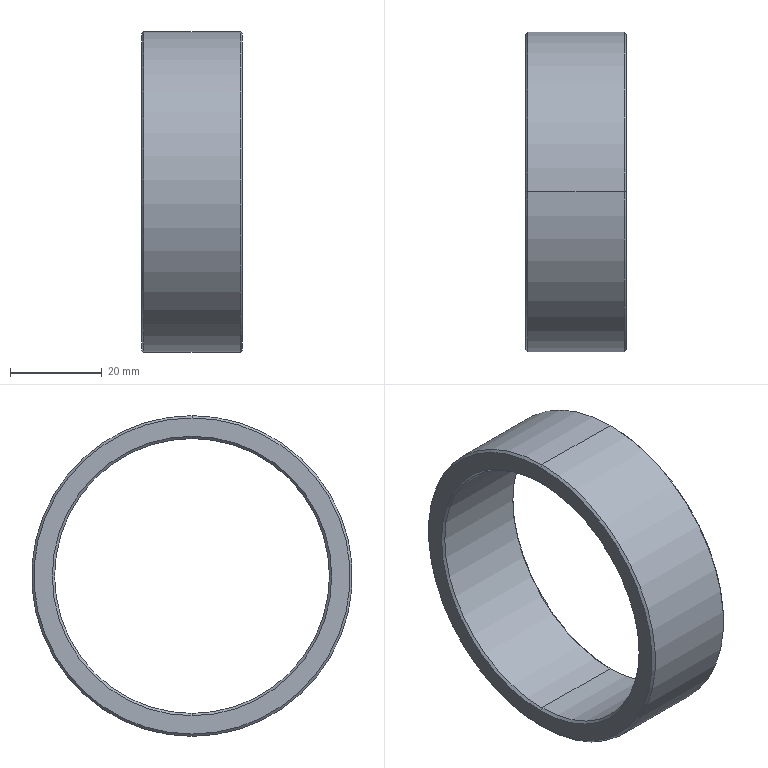Component | SolidWorks | Oil-impregnatedBushing-1 | 1 solid | 14 faces | box 22 x 70 x 70 mm | volume 22360 mm3 | cone 8 | cylinder 4 | plane 2 | commonest cylinder face diameters 60 x2 70 x2
build123d program:
from build123d import *

# Parameters (mm, degrees)
SKETCH1_R           = 35
SKETCH1_R_2         = 30
BOSS_EXTRUDE1_DEPTH = 22
CHAMFER1_SIZE       = 0.5


with BuildPart() as part:
    # Sketch1 → Boss-Extrude1 (new body)
    with BuildSketch(Plane.XY):
        Circle(SKETCH1_R)
        Circle(SKETCH1_R_2, mode=Mode.SUBTRACT)
    extrude(amount=BOSS_EXTRUDE1_DEPTH)

    # Chamfer1
    chamfer1_edges = [part.edges().sort_by_distance(p)[0] for p in [
        (-35, 0, 0),
        (-35, 0, 22),
        (-30, 0, 0),
        (-30, 0, 22),
    ]]
    chamfer(chamfer1_edges, length=CHAMFER1_SIZE)


solid = part.part

# Placed as in the assembly
solid = solid.moved(Location((-477.809, 275.819, 0), (0, 90, 0)))
STEP:
#1=COLOUR_RGB('',0.7922,0.8196,0.9333);
#2=FILL_AREA_STYLE_COLOUR('',#1);
#3=FILL_AREA_STYLE('',(#2));
#4=SURFACE_STYLE_FILL_AREA(#3);
#5=SURFACE_SIDE_STYLE('',(#4));
#6=SURFACE_STYLE_USAGE(.BOTH.,#5);
#7=PRESENTATION_STYLE_ASSIGNMENT((#6));
#8=CARTESIAN_POINT('',(-17.965,10.859,1.181));
#9=VERTEX_POINT('',#8);
#10=CARTESIAN_POINT('',(-17.965,10.859,-1.181));
#11=VERTEX_POINT('',#10);
#12=CARTESIAN_POINT('',(-17.965,10.859,0.));
#13=DIRECTION('',(1.,0.,0.));
#14=DIRECTION('',(0.,0.,-1.));
#15=AXIS2_PLACEMENT_3D('',#12,#13,#14);
#16=CIRCLE('',#15,1.181);
#17=EDGE_CURVE('',#9,#11,#16,.T.);
#18=ORIENTED_EDGE('',*,*,#17,.F.);
#19=CARTESIAN_POINT('',(-17.945,10.859,1.201));
#20=VERTEX_POINT('',#19);
#21=CARTESIAN_POINT('',(-17.965,10.859,1.181));
#22=DIRECTION('',(0.7071,0.,0.7071));
#23=VECTOR('',#22,39.37);
#24=LINE('',#21,#23);
#25=EDGE_CURVE('',#9,#20,#24,.T.);
#26=ORIENTED_EDGE('',*,*,#25,.T.);
#27=CARTESIAN_POINT('',(-17.945,10.859,-1.201));
#28=VERTEX_POINT('',#27);
#29=CARTESIAN_POINT('',(-17.945,10.859,0.));
#30=DIRECTION('',(-1.,0.,0.));
#31=DIRECTION('',(0.,0.,-1.));
#32=AXIS2_PLACEMENT_3D('',#29,#30,#31);
#33=CIRCLE('',#32,1.201);
#34=EDGE_CURVE('',#28,#20,#33,.T.);
#35=ORIENTED_EDGE('',*,*,#34,.F.);
#36=CARTESIAN_POINT('',(-17.965,10.859,-1.181));
#37=DIRECTION('',(0.7071,0.,-0.7071));
#38=VECTOR('',#37,39.37);
#39=LINE('',#36,#38);
#40=EDGE_CURVE('',#11,#28,#39,.T.);
#41=ORIENTED_EDGE('',*,*,#40,.F.);
#42=EDGE_LOOP('',(#18,#26,#35,#41));
#43=FACE_OUTER_BOUND('',#42,.T.);
#44=CARTESIAN_POINT('',(-17.965,10.859,0.));
#45=DIRECTION('',(1.,0.,0.));
#46=DIRECTION('',(0.,0.,-1.));
#47=AXIS2_PLACEMENT_3D('',#44,#45,#46);
#48=CONICAL_SURFACE('',#47,1.181,0.7854);
#49=ADVANCED_FACE('',(#43),#48,.F.);
#50=CARTESIAN_POINT('',(-17.945,10.859,-1.358));
#51=VERTEX_POINT('',#50);
#52=CARTESIAN_POINT('',(-17.945,10.859,1.358));
#53=VERTEX_POINT('',#52);
#54=CARTESIAN_POINT('',(-17.945,10.859,0.));
#55=DIRECTION('',(1.,0.,0.));
#56=DIRECTION('',(0.,0.,-1.));
#57=AXIS2_PLACEMENT_3D('',#54,#55,#56);
#58=CIRCLE('',#57,1.358);
#59=EDGE_CURVE('',#51,#53,#58,.T.);
#60=ORIENTED_EDGE('',*,*,#59,.F.);
#61=CARTESIAN_POINT('',(-17.965,10.859,-1.378));
#62=VERTEX_POINT('',#61);
#63=CARTESIAN_POINT('',(-17.945,10.859,-1.358));
#64=DIRECTION('',(-0.7071,0.,-0.7071));
#65=VECTOR('',#64,39.37);
#66=LINE('',#63,#65);
#67=EDGE_CURVE('',#51,#62,#66,.T.);
#68=ORIENTED_EDGE('',*,*,#67,.T.);
#69=CARTESIAN_POINT('',(-17.965,10.859,1.378));
#70=VERTEX_POINT('',#69);
#71=CARTESIAN_POINT('',(-17.965,10.859,0.));
#72=DIRECTION('',(-1.,0.,0.));
#73=DIRECTION('',(0.,0.,-1.));
#74=AXIS2_PLACEMENT_3D('',#71,#72,#73);
#75=CIRCLE('',#74,1.378);
#76=EDGE_CURVE('',#70,#62,#75,.T.);
#77=ORIENTED_EDGE('',*,*,#76,.F.);
#78=CARTESIAN_POINT('',(-17.945,10.859,1.358));
#79=DIRECTION('',(-0.7071,0.,0.7071));
#80=VECTOR('',#79,39.37);
#81=LINE('',#78,#80);
#82=EDGE_CURVE('',#53,#70,#81,.T.);
#83=ORIENTED_EDGE('',*,*,#82,.F.);
#84=EDGE_LOOP('',(#60,#68,#77,#83));
#85=FACE_OUTER_BOUND('',#84,.T.);
#86=CARTESIAN_POINT('',(-17.945,10.859,0.));
#87=DIRECTION('',(-1.,0.,0.));
#88=DIRECTION('',(0.,0.,1.));
#89=AXIS2_PLACEMENT_3D('',#86,#87,#88);
#90=CONICAL_SURFACE('',#89,1.358,0.7854);
#91=ADVANCED_FACE('',(#85),#90,.T.);
#92=CARTESIAN_POINT('',(-18.792,10.859,-1.181));
#93=VERTEX_POINT('',#92);
#94=CARTESIAN_POINT('',(-18.792,10.859,1.181));
#95=VERTEX_POINT('',#94);
#96=CARTESIAN_POINT('',(-18.792,10.859,0.));
#97=DIRECTION('',(-1.,0.,0.));
#98=DIRECTION('',(0.,0.,-1.));
#99=AXIS2_PLACEMENT_3D('',#96,#97,#98);
#100=CIRCLE('',#99,1.181);
#101=EDGE_CURVE('',#93,#95,#100,.T.);
#102=ORIENTED_EDGE('',*,*,#101,.F.);
#103=CARTESIAN_POINT('',(-18.811,10.859,-1.201));
#104=VERTEX_POINT('',#103);
#105=CARTESIAN_POINT('',(-18.811,10.859,-1.201));
#106=DIRECTION('',(-0.7071,0.,-0.7071));
#107=VECTOR('',#106,39.37);
#108=LINE('',#105,#107);
#109=EDGE_CURVE('',#93,#104,#108,.T.);
#110=ORIENTED_EDGE('',*,*,#109,.T.);
#111=CARTESIAN_POINT('',(-18.811,10.859,1.201));
#112=VERTEX_POINT('',#111);
#113=CARTESIAN_POINT('',(-18.811,10.859,0.));
#114=DIRECTION('',(1.,0.,0.));
#115=DIRECTION('',(0.,0.,-1.));
#116=AXIS2_PLACEMENT_3D('',#113,#114,#115);
#117=CIRCLE('',#116,1.201);
#118=EDGE_CURVE('',#112,#104,#117,.T.);
#119=ORIENTED_EDGE('',*,*,#118,.F.);
#120=CARTESIAN_POINT('',(-18.811,10.859,1.201));
#121=DIRECTION('',(-0.7071,0.,0.7071));
#122=VECTOR('',#121,39.37);
#123=LINE('',#120,#122);
#124=EDGE_CURVE('',#95,#112,#123,.T.);
#125=ORIENTED_EDGE('',*,*,#124,.F.);
#126=EDGE_LOOP('',(#102,#110,#119,#125));
#127=FACE_OUTER_BOUND('',#126,.T.);
#128=CARTESIAN_POINT('',(-18.811,10.859,0.));
#129=DIRECTION('',(-1.,0.,0.));
#130=DIRECTION('',(0.,0.,1.));
#131=AXIS2_PLACEMENT_3D('',#128,#129,#130);
#132=CONICAL_SURFACE('',#131,1.201,0.7854);
#133=ADVANCED_FACE('',(#127),#132,.F.);
#134=CARTESIAN_POINT('',(-18.811,10.859,1.358));
#135=VERTEX_POINT('',#134);
#136=CARTESIAN_POINT('',(-18.811,10.859,-1.358));
#137=VERTEX_POINT('',#136);
#138=CARTESIAN_POINT('',(-18.811,10.859,0.));
#139=DIRECTION('',(-1.,0.,0.));
#140=DIRECTION('',(0.,0.,-1.));
#141=AXIS2_PLACEMENT_3D('',#138,#139,#140);
#142=CIRCLE('',#141,1.358);
#143=EDGE_CURVE('',#135,#137,#142,.T.);
#144=ORIENTED_EDGE('',*,*,#143,.F.);
#145=CARTESIAN_POINT('',(-18.792,10.859,1.378));
#146=VERTEX_POINT('',#145);
#147=CARTESIAN_POINT('',(-18.792,10.859,1.378));
#148=DIRECTION('',(0.7071,0.,0.7071));
#149=VECTOR('',#148,39.37);
#150=LINE('',#147,#149);
#151=EDGE_CURVE('',#135,#146,#150,.T.);
#152=ORIENTED_EDGE('',*,*,#151,.T.);
#153=CARTESIAN_POINT('',(-18.792,10.859,-1.378));
#154=VERTEX_POINT('',#153);
#155=CARTESIAN_POINT('',(-18.792,10.859,0.));
#156=DIRECTION('',(1.,0.,0.));
#157=DIRECTION('',(0.,0.,-1.));
#158=AXIS2_PLACEMENT_3D('',#155,#156,#157);
#159=CIRCLE('',#158,1.378);
#160=EDGE_CURVE('',#154,#146,#159,.T.);
#161=ORIENTED_EDGE('',*,*,#160,.F.);
#162=CARTESIAN_POINT('',(-18.792,10.859,-1.378));
#163=DIRECTION('',(0.7071,0.,-0.7071));
#164=VECTOR('',#163,39.37);
#165=LINE('',#162,#164);
#166=EDGE_CURVE('',#137,#154,#165,.T.);
#167=ORIENTED_EDGE('',*,*,#166,.F.);
#168=EDGE_LOOP('',(#144,#152,#161,#167));
#169=FACE_OUTER_BOUND('',#168,.T.);
#170=CARTESIAN_POINT('',(-18.792,10.859,0.));
#171=DIRECTION('',(1.,0.,0.));
#172=DIRECTION('',(0.,0.,-1.));
#173=AXIS2_PLACEMENT_3D('',#170,#171,#172);
#174=CONICAL_SURFACE('',#173,1.378,0.7854);
#175=ADVANCED_FACE('',(#169),#174,.T.);
#176=ORIENTED_EDGE('',*,*,#17,.T.);
#177=CARTESIAN_POINT('',(-17.945,10.859,-1.181));
#178=DIRECTION('',(-1.,0.,0.));
#179=VECTOR('',#178,39.37);
#180=LINE('',#177,#179);
#181=EDGE_CURVE('',#11,#93,#180,.T.);
#182=ORIENTED_EDGE('',*,*,#181,.T.);
#183=ORIENTED_EDGE('',*,*,#101,.T.);
#184=CARTESIAN_POINT('',(-17.945,10.859,1.181));
#185=DIRECTION('',(-1.,0.,0.));
#186=VECTOR('',#185,39.37);
#187=LINE('',#184,#186);
#188=EDGE_CURVE('',#9,#95,#187,.T.);
#189=ORIENTED_EDGE('',*,*,#188,.F.);
#190=EDGE_LOOP('',(#176,#182,#183,#189));
#191=FACE_OUTER_BOUND('',#190,.T.);
#192=CARTESIAN_POINT('',(-17.945,10.859,0.));
#193=DIRECTION('',(-1.,0.,0.));
#194=DIRECTION('',(0.,0.,1.));
#195=AXIS2_PLACEMENT_3D('',#192,#193,#194);
#196=CYLINDRICAL_SURFACE('',#195,1.181);
#197=ADVANCED_FACE('',(#191),#196,.F.);
#198=ORIENTED_EDGE('',*,*,#76,.T.);
#199=CARTESIAN_POINT('',(-17.945,10.859,-1.378));
#200=DIRECTION('',(-1.,0.,0.));
#201=VECTOR('',#200,39.37);
#202=LINE('',#199,#201);
#203=EDGE_CURVE('',#62,#154,#202,.T.);
#204=ORIENTED_EDGE('',*,*,#203,.T.);
#205=ORIENTED_EDGE('',*,*,#160,.T.);
#206=CARTESIAN_POINT('',(-17.945,10.859,1.378));
#207=DIRECTION('',(-1.,0.,0.));
#208=VECTOR('',#207,39.37);
#209=LINE('',#206,#208);
#210=EDGE_CURVE('',#70,#146,#209,.T.);
#211=ORIENTED_EDGE('',*,*,#210,.F.);
#212=EDGE_LOOP('',(#198,#204,#205,#211));
#213=FACE_OUTER_BOUND('',#212,.T.);
#214=CARTESIAN_POINT('',(-17.945,10.859,0.));
#215=DIRECTION('',(-1.,0.,0.));
#216=DIRECTION('',(0.,0.,1.));
#217=AXIS2_PLACEMENT_3D('',#214,#215,#216);
#218=CYLINDRICAL_SURFACE('',#217,1.378);
#219=ADVANCED_FACE('',(#213),#218,.T.);
#220=CARTESIAN_POINT('',(-17.945,10.859,0.));
#221=DIRECTION('',(1.,0.,0.));
#222=DIRECTION('',(0.,0.,-1.));
#223=AXIS2_PLACEMENT_3D('',#220,#221,#222);
#224=CIRCLE('',#223,1.358);
#225=EDGE_CURVE('',#53,#51,#224,.T.);
#226=ORIENTED_EDGE('',*,*,#225,.T.);
#227=ORIENTED_EDGE('',*,*,#59,.T.);
#228=EDGE_LOOP('',(#226,#227));
#229=FACE_OUTER_BOUND('',#228,.T.);
#230=ORIENTED_EDGE('',*,*,#34,.T.);
#231=CARTESIAN_POINT('',(-17.945,10.859,0.));
#232=DIRECTION('',(-1.,0.,0.));
#233=DIRECTION('',(0.,0.,-1.));
#234=AXIS2_PLACEMENT_3D('',#231,#232,#233);
#235=CIRCLE('',#234,1.201);
#236=EDGE_CURVE('',#20,#28,#235,.T.);
#237=ORIENTED_EDGE('',*,*,#236,.T.);
#238=EDGE_LOOP('',(#230,#237));
#239=FACE_BOUND('',#238,.T.);
#240=CARTESIAN_POINT('',(-17.945,10.859,0.));
#241=DIRECTION('',(1.,0.,0.));
#242=DIRECTION('',(0.,0.,-1.));
#243=AXIS2_PLACEMENT_3D('',#240,#241,#242);
#244=PLANE('',#243);
#245=ADVANCED_FACE('',(#229,#239),#244,.T.);
#246=CARTESIAN_POINT('',(-18.811,10.859,0.));
#247=DIRECTION('',(-1.,0.,0.));
#248=DIRECTION('',(0.,0.,-1.));
#249=AXIS2_PLACEMENT_3D('',#246,#247,#248);
#250=CIRCLE('',#249,1.358);
#251=EDGE_CURVE('',#137,#135,#250,.T.);
#252=ORIENTED_EDGE('',*,*,#251,.T.);
#253=ORIENTED_EDGE('',*,*,#143,.T.);
#254=EDGE_LOOP('',(#252,#253));
#255=FACE_OUTER_BOUND('',#254,.T.);
#256=ORIENTED_EDGE('',*,*,#118,.T.);
#257=CARTESIAN_POINT('',(-18.811,10.859,0.));
#258=DIRECTION('',(1.,0.,0.));
#259=DIRECTION('',(0.,0.,-1.));
#260=AXIS2_PLACEMENT_3D('',#257,#258,#259);
#261=CIRCLE('',#260,1.201);
#262=EDGE_CURVE('',#104,#112,#261,.T.);
#263=ORIENTED_EDGE('',*,*,#262,.T.);
#264=EDGE_LOOP('',(#256,#263));
#265=FACE_BOUND('',#264,.T.);
#266=CARTESIAN_POINT('',(-18.811,10.859,0.));
#267=DIRECTION('',(1.,0.,0.));
#268=DIRECTION('',(0.,0.,-1.));
#269=AXIS2_PLACEMENT_3D('',#266,#267,#268);
#270=PLANE('',#269);
#271=ADVANCED_FACE('',(#255,#265),#270,.F.);
#272=ORIENTED_EDGE('',*,*,#203,.F.);
#273=CARTESIAN_POINT('',(-17.965,10.859,0.));
#274=DIRECTION('',(-1.,0.,0.));
#275=DIRECTION('',(0.,0.,-1.));
#276=AXIS2_PLACEMENT_3D('',#273,#274,#275);
#277=CIRCLE('',#276,1.378);
#278=EDGE_CURVE('',#62,#70,#277,.T.);
#279=ORIENTED_EDGE('',*,*,#278,.T.);
#280=ORIENTED_EDGE('',*,*,#210,.T.);
#281=CARTESIAN_POINT('',(-18.792,10.859,0.));
#282=DIRECTION('',(1.,0.,0.));
#283=DIRECTION('',(0.,0.,-1.));
#284=AXIS2_PLACEMENT_3D('',#281,#282,#283);
#285=CIRCLE('',#284,1.378);
#286=EDGE_CURVE('',#146,#154,#285,.T.);
#287=ORIENTED_EDGE('',*,*,#286,.T.);
#288=EDGE_LOOP('',(#272,#279,#280,#287));
#289=FACE_OUTER_BOUND('',#288,.T.);
#290=CARTESIAN_POINT('',(-17.945,10.859,0.));
#291=DIRECTION('',(-1.,0.,0.));
#292=DIRECTION('',(0.,0.,1.));
#293=AXIS2_PLACEMENT_3D('',#290,#291,#292);
#294=CYLINDRICAL_SURFACE('',#293,1.378);
#295=ADVANCED_FACE('',(#289),#294,.T.);
#296=ORIENTED_EDGE('',*,*,#181,.F.);
#297=CARTESIAN_POINT('',(-17.965,10.859,0.));
#298=DIRECTION('',(1.,0.,0.));
#299=DIRECTION('',(0.,0.,-1.));
#300=AXIS2_PLACEMENT_3D('',#297,#298,#299);
#301=CIRCLE('',#300,1.181);
#302=EDGE_CURVE('',#11,#9,#301,.T.);
#303=ORIENTED_EDGE('',*,*,#302,.T.);
#304=ORIENTED_EDGE('',*,*,#188,.T.);
#305=CARTESIAN_POINT('',(-18.792,10.859,0.));
#306=DIRECTION('',(-1.,0.,0.));
#307=DIRECTION('',(0.,0.,-1.));
#308=AXIS2_PLACEMENT_3D('',#305,#306,#307);
#309=CIRCLE('',#308,1.181);
#310=EDGE_CURVE('',#95,#93,#309,.T.);
#311=ORIENTED_EDGE('',*,*,#310,.T.);
#312=EDGE_LOOP('',(#296,#303,#304,#311));
#313=FACE_OUTER_BOUND('',#312,.T.);
#314=CARTESIAN_POINT('',(-17.945,10.859,0.));
#315=DIRECTION('',(-1.,0.,0.));
#316=DIRECTION('',(0.,0.,1.));
#317=AXIS2_PLACEMENT_3D('',#314,#315,#316);
#318=CYLINDRICAL_SURFACE('',#317,1.181);
#319=ADVANCED_FACE('',(#313),#318,.F.);
#320=ORIENTED_EDGE('',*,*,#151,.F.);
#321=ORIENTED_EDGE('',*,*,#251,.F.);
#322=ORIENTED_EDGE('',*,*,#166,.T.);
#323=ORIENTED_EDGE('',*,*,#286,.F.);
#324=EDGE_LOOP('',(#320,#321,#322,#323));
#325=FACE_OUTER_BOUND('',#324,.T.);
#326=CARTESIAN_POINT('',(-18.792,10.859,0.));
#327=DIRECTION('',(1.,0.,0.));
#328=DIRECTION('',(0.,0.,-1.));
#329=AXIS2_PLACEMENT_3D('',#326,#327,#328);
#330=CONICAL_SURFACE('',#329,1.378,0.7854);
#331=ADVANCED_FACE('',(#325),#330,.T.);
#332=ORIENTED_EDGE('',*,*,#109,.F.);
#333=ORIENTED_EDGE('',*,*,#310,.F.);
#334=ORIENTED_EDGE('',*,*,#124,.T.);
#335=ORIENTED_EDGE('',*,*,#262,.F.);
#336=EDGE_LOOP('',(#332,#333,#334,#335));
#337=FACE_OUTER_BOUND('',#336,.T.);
#338=CARTESIAN_POINT('',(-18.811,10.859,0.));
#339=DIRECTION('',(-1.,0.,0.));
#340=DIRECTION('',(0.,0.,1.));
#341=AXIS2_PLACEMENT_3D('',#338,#339,#340);
#342=CONICAL_SURFACE('',#341,1.201,0.7854);
#343=ADVANCED_FACE('',(#337),#342,.F.);
#344=ORIENTED_EDGE('',*,*,#67,.F.);
#345=ORIENTED_EDGE('',*,*,#225,.F.);
#346=ORIENTED_EDGE('',*,*,#82,.T.);
#347=ORIENTED_EDGE('',*,*,#278,.F.);
#348=EDGE_LOOP('',(#344,#345,#346,#347));
#349=FACE_OUTER_BOUND('',#348,.T.);
#350=CARTESIAN_POINT('',(-17.945,10.859,0.));
#351=DIRECTION('',(-1.,0.,0.));
#352=DIRECTION('',(0.,0.,1.));
#353=AXIS2_PLACEMENT_3D('',#350,#351,#352);
#354=CONICAL_SURFACE('',#353,1.358,0.7854);
#355=ADVANCED_FACE('',(#349),#354,.T.);
#356=ORIENTED_EDGE('',*,*,#25,.F.);
#357=ORIENTED_EDGE('',*,*,#302,.F.);
#358=ORIENTED_EDGE('',*,*,#40,.T.);
#359=ORIENTED_EDGE('',*,*,#236,.F.);
#360=EDGE_LOOP('',(#356,#357,#358,#359));
#361=FACE_OUTER_BOUND('',#360,.T.);
#362=CARTESIAN_POINT('',(-17.965,10.859,0.));
#363=DIRECTION('',(1.,0.,0.));
#364=DIRECTION('',(0.,0.,-1.));
#365=AXIS2_PLACEMENT_3D('',#362,#363,#364);
#366=CONICAL_SURFACE('',#365,1.181,0.7854);
#367=ADVANCED_FACE('',(#361),#366,.F.);
#368=CLOSED_SHELL('',(#49,#91,#133,#175,#197,#219,#245,#271,#295,#319,#331,#343,#355,#367));
#369=MANIFOLD_SOLID_BREP('',#368);
#370=STYLED_ITEM('',(#7),#369);
#371=(LENGTH_UNIT()NAMED_UNIT(*)SI_UNIT($,.METRE.));
#372=LENGTH_MEASURE_WITH_UNIT(LENGTH_MEASURE(0.0254),#371);
#373=DIMENSIONAL_EXPONENTS(1.,0.,0.,0.,0.,0.,0.);
#374=(CONVERSION_BASED_UNIT('',#372)LENGTH_UNIT()NAMED_UNIT(#373));
#375=UNCERTAINTY_MEASURE_WITH_UNIT(LENGTH_MEASURE(0.00001),#374,'','');
#376=(NAMED_UNIT(*)PLANE_ANGLE_UNIT()SI_UNIT($,.RADIAN.));
#377=(NAMED_UNIT(*)SI_UNIT($,.STERADIAN.)SOLID_ANGLE_UNIT());
#378=(GEOMETRIC_REPRESENTATION_CONTEXT(3)GLOBAL_UNCERTAINTY_ASSIGNED_CONTEXT((#375))GLOBAL_UNIT_ASSIGNED_CONTEXT((#374,#376,#377))REPRESENTATION_CONTEXT('',''));
#379=MECHANICAL_DESIGN_GEOMETRIC_PRESENTATION_REPRESENTATION('',(#370),#378);
#380=PRESENTATION_LAYER_ASSIGNMENT('','',(#370));
#381=CARTESIAN_POINT('',(0.,0.,0.));
#382=DIRECTION('',(0.,0.,1.));
#383=DIRECTION('',(1.,0.,0.));
#384=AXIS2_PLACEMENT_3D('',#381,#382,#383);
#385=(LENGTH_UNIT()NAMED_UNIT(*)SI_UNIT($,.METRE.));
#386=LENGTH_MEASURE_WITH_UNIT(LENGTH_MEASURE(0.0254),#385);
#387=DIMENSIONAL_EXPONENTS(1.,0.,0.,0.,0.,0.,0.);
#388=(CONVERSION_BASED_UNIT('',#386)LENGTH_UNIT()NAMED_UNIT(#387));
#389=UNCERTAINTY_MEASURE_WITH_UNIT(LENGTH_MEASURE(0.00001),#388,'','');
#390=(NAMED_UNIT(*)PLANE_ANGLE_UNIT()SI_UNIT($,.RADIAN.));
#391=(NAMED_UNIT(*)SI_UNIT($,.STERADIAN.)SOLID_ANGLE_UNIT());
#392=(GEOMETRIC_REPRESENTATION_CONTEXT(3)GLOBAL_UNCERTAINTY_ASSIGNED_CONTEXT((#389))GLOBAL_UNIT_ASSIGNED_CONTEXT((#388,#390,#391))REPRESENTATION_CONTEXT('',''));
#393=ADVANCED_BREP_SHAPE_REPRESENTATION('',(#369,#384),#392);